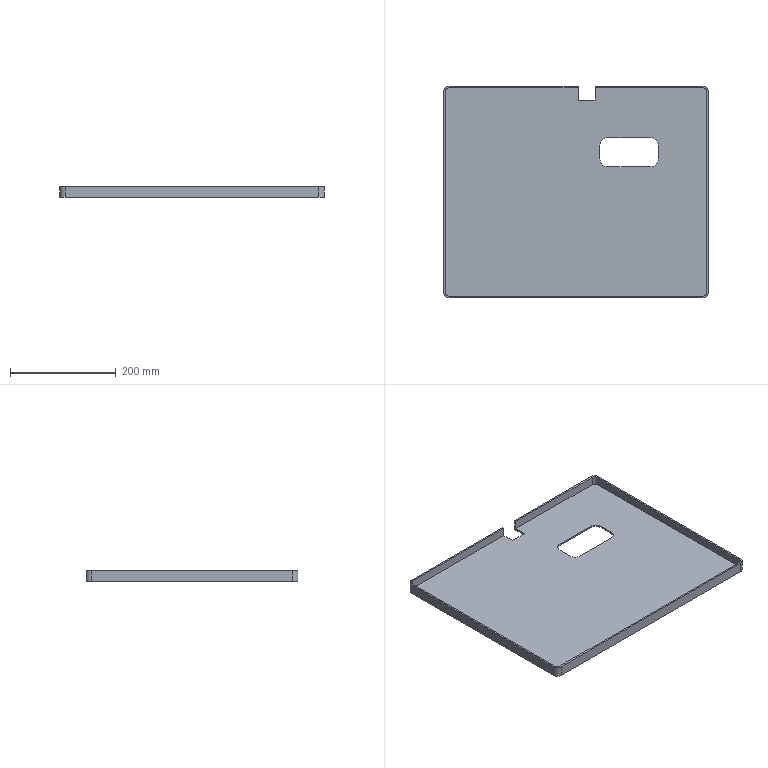Component | SolidWorks | LX-TSJ-16-2 | 1 solid | 32 faces | box 500 x 400 x 20 mm | volume 668381 mm3 | plane 20 | cylinder 12 | commonest cylinder face diameters 20 x4 14 x4 30 x4
STEP:
#1=COLOUR_RGB('',0.7922,0.8196,0.9333);
#2=FILL_AREA_STYLE_COLOUR('',#1);
#3=FILL_AREA_STYLE('',(#2));
#4=SURFACE_STYLE_FILL_AREA(#3);
#5=SURFACE_SIDE_STYLE('',(#4));
#6=SURFACE_STYLE_USAGE(.BOTH.,#5);
#7=PRESENTATION_STYLE_ASSIGNMENT((#6));
#8=CARTESIAN_POINT('',(-5.473,-15.275,-26.153));
#9=VERTEX_POINT('',#8);
#10=CARTESIAN_POINT('',(-5.473,-15.275,-26.823));
#11=VERTEX_POINT('',#10);
#12=CARTESIAN_POINT('',(-5.473,-15.275,-26.153));
#13=DIRECTION('',(0.,0.,-1.));
#14=VECTOR('',#13,39.37);
#15=LINE('',#12,#14);
#16=EDGE_CURVE('',#9,#11,#15,.T.);
#17=ORIENTED_EDGE('',*,*,#16,.F.);
#18=CARTESIAN_POINT('',(-15.08,-15.275,-26.153));
#19=VERTEX_POINT('',#18);
#20=CARTESIAN_POINT('',(-15.08,-15.275,-26.153));
#21=DIRECTION('',(1.,0.,0.));
#22=VECTOR('',#21,39.37);
#23=LINE('',#20,#22);
#24=EDGE_CURVE('',#19,#9,#23,.T.);
#25=ORIENTED_EDGE('',*,*,#24,.F.);
#26=CARTESIAN_POINT('',(-15.08,-15.275,-26.823));
#27=VERTEX_POINT('',#26);
#28=CARTESIAN_POINT('',(-15.08,-15.275,-26.153));
#29=DIRECTION('',(0.,0.,-1.));
#30=VECTOR('',#29,39.37);
#31=LINE('',#28,#30);
#32=EDGE_CURVE('',#19,#27,#31,.T.);
#33=ORIENTED_EDGE('',*,*,#32,.T.);
#34=CARTESIAN_POINT('',(-15.08,-15.275,-26.823));
#35=DIRECTION('',(1.,0.,0.));
#36=VECTOR('',#35,39.37);
#37=LINE('',#34,#36);
#38=EDGE_CURVE('',#27,#11,#37,.T.);
#39=ORIENTED_EDGE('',*,*,#38,.T.);
#40=EDGE_LOOP('',(#17,#25,#33,#39));
#41=FACE_OUTER_BOUND('',#40,.T.);
#42=CARTESIAN_POINT('',(-15.08,-15.275,-26.153));
#43=DIRECTION('',(0.,-1.,0.));
#44=DIRECTION('',(0.,0.,-1.));
#45=AXIS2_PLACEMENT_3D('',#42,#43,#44);
#46=PLANE('',#45);
#47=ADVANCED_FACE('',(#41),#46,.T.);
#48=CARTESIAN_POINT('',(-5.473,-15.157,-26.153));
#49=VERTEX_POINT('',#48);
#50=CARTESIAN_POINT('',(-15.08,-15.157,-26.153));
#51=VERTEX_POINT('',#50);
#52=CARTESIAN_POINT('',(-15.08,-15.157,-26.153));
#53=DIRECTION('',(-1.,0.,0.));
#54=VECTOR('',#53,39.37);
#55=LINE('',#52,#54);
#56=EDGE_CURVE('',#49,#51,#55,.T.);
#57=ORIENTED_EDGE('',*,*,#56,.F.);
#58=CARTESIAN_POINT('',(-5.473,-15.157,-26.941));
#59=VERTEX_POINT('',#58);
#60=CARTESIAN_POINT('',(-5.473,-15.157,-26.153));
#61=DIRECTION('',(0.,0.,-1.));
#62=VECTOR('',#61,39.37);
#63=LINE('',#60,#62);
#64=EDGE_CURVE('',#49,#59,#63,.T.);
#65=ORIENTED_EDGE('',*,*,#64,.T.);
#66=CARTESIAN_POINT('',(-15.08,-15.157,-26.941));
#67=VERTEX_POINT('',#66);
#68=CARTESIAN_POINT('',(-15.08,-15.157,-26.941));
#69=DIRECTION('',(-1.,0.,0.));
#70=VECTOR('',#69,39.37);
#71=LINE('',#68,#70);
#72=EDGE_CURVE('',#59,#67,#71,.T.);
#73=ORIENTED_EDGE('',*,*,#72,.T.);
#74=CARTESIAN_POINT('',(-15.08,-15.157,-26.153));
#75=DIRECTION('',(0.,0.,-1.));
#76=VECTOR('',#75,39.37);
#77=LINE('',#74,#76);
#78=EDGE_CURVE('',#51,#67,#77,.T.);
#79=ORIENTED_EDGE('',*,*,#78,.F.);
#80=EDGE_LOOP('',(#57,#65,#73,#79));
#81=FACE_OUTER_BOUND('',#80,.T.);
#82=CARTESIAN_POINT('',(-15.08,-15.157,-26.153));
#83=DIRECTION('',(0.,-1.,0.));
#84=DIRECTION('',(0.,0.,-1.));
#85=AXIS2_PLACEMENT_3D('',#82,#83,#84);
#86=PLANE('',#85);
#87=ADVANCED_FACE('',(#81),#86,.F.);
#88=ORIENTED_EDGE('',*,*,#72,.F.);
#89=CARTESIAN_POINT('',(-5.473,-16.18,-26.941));
#90=VERTEX_POINT('',#89);
#91=CARTESIAN_POINT('',(-5.473,-30.511,-26.941));
#92=DIRECTION('',(0.,-1.,0.));
#93=VECTOR('',#92,39.37);
#94=LINE('',#91,#93);
#95=EDGE_CURVE('',#59,#90,#94,.T.);
#96=ORIENTED_EDGE('',*,*,#95,.T.);
#97=CARTESIAN_POINT('',(-4.213,-16.18,-26.941));
#98=VERTEX_POINT('',#97);
#99=CARTESIAN_POINT('',(-15.08,-16.18,-26.941));
#100=DIRECTION('',(1.,0.,0.));
#101=VECTOR('',#100,39.37);
#102=LINE('',#99,#101);
#103=EDGE_CURVE('',#90,#98,#102,.T.);
#104=ORIENTED_EDGE('',*,*,#103,.T.);
#105=CARTESIAN_POINT('',(-4.213,-15.157,-26.941));
#106=VERTEX_POINT('',#105);
#107=CARTESIAN_POINT('',(-4.213,-30.511,-26.941));
#108=DIRECTION('',(0.,1.,0.));
#109=VECTOR('',#108,39.37);
#110=LINE('',#107,#109);
#111=EDGE_CURVE('',#98,#106,#110,.T.);
#112=ORIENTED_EDGE('',*,*,#111,.T.);
#113=CARTESIAN_POINT('',(3.818,-15.157,-26.941));
#114=VERTEX_POINT('',#113);
#115=CARTESIAN_POINT('',(-15.08,-15.157,-26.941));
#116=DIRECTION('',(-1.,0.,0.));
#117=VECTOR('',#116,39.37);
#118=LINE('',#115,#117);
#119=EDGE_CURVE('',#114,#106,#118,.T.);
#120=ORIENTED_EDGE('',*,*,#119,.F.);
#121=CARTESIAN_POINT('',(4.212,-15.55,-26.941));
#122=VERTEX_POINT('',#121);
#123=CARTESIAN_POINT('',(3.818,-15.55,-26.941));
#124=DIRECTION('',(0.,0.,1.));
#125=DIRECTION('',(-1.,0.,0.));
#126=AXIS2_PLACEMENT_3D('',#123,#124,#125);
#127=CIRCLE('',#126,0.3937);
#128=EDGE_CURVE('',#122,#114,#127,.T.);
#129=ORIENTED_EDGE('',*,*,#128,.F.);
#130=CARTESIAN_POINT('',(4.212,-30.511,-26.941));
#131=VERTEX_POINT('',#130);
#132=CARTESIAN_POINT('',(4.212,-30.511,-26.941));
#133=DIRECTION('',(0.,1.,0.));
#134=VECTOR('',#133,39.37);
#135=LINE('',#132,#134);
#136=EDGE_CURVE('',#131,#122,#135,.T.);
#137=ORIENTED_EDGE('',*,*,#136,.F.);
#138=CARTESIAN_POINT('',(3.818,-30.905,-26.941));
#139=VERTEX_POINT('',#138);
#140=CARTESIAN_POINT('',(3.818,-30.511,-26.941));
#141=DIRECTION('',(0.,0.,1.));
#142=DIRECTION('',(-1.,0.,0.));
#143=AXIS2_PLACEMENT_3D('',#140,#141,#142);
#144=CIRCLE('',#143,0.3937);
#145=EDGE_CURVE('',#139,#131,#144,.T.);
#146=ORIENTED_EDGE('',*,*,#145,.F.);
#147=CARTESIAN_POINT('',(-15.08,-30.905,-26.941));
#148=VERTEX_POINT('',#147);
#149=CARTESIAN_POINT('',(-15.08,-30.905,-26.941));
#150=DIRECTION('',(1.,0.,0.));
#151=VECTOR('',#150,39.37);
#152=LINE('',#149,#151);
#153=EDGE_CURVE('',#148,#139,#152,.T.);
#154=ORIENTED_EDGE('',*,*,#153,.F.);
#155=CARTESIAN_POINT('',(-15.473,-30.511,-26.941));
#156=VERTEX_POINT('',#155);
#157=CARTESIAN_POINT('',(-15.08,-30.511,-26.941));
#158=DIRECTION('',(0.,0.,1.));
#159=DIRECTION('',(-1.,0.,0.));
#160=AXIS2_PLACEMENT_3D('',#157,#158,#159);
#161=CIRCLE('',#160,0.3937);
#162=EDGE_CURVE('',#156,#148,#161,.T.);
#163=ORIENTED_EDGE('',*,*,#162,.F.);
#164=CARTESIAN_POINT('',(-15.473,-15.55,-26.941));
#165=VERTEX_POINT('',#164);
#166=CARTESIAN_POINT('',(-15.473,-30.511,-26.941));
#167=DIRECTION('',(0.,-1.,0.));
#168=VECTOR('',#167,39.37);
#169=LINE('',#166,#168);
#170=EDGE_CURVE('',#165,#156,#169,.T.);
#171=ORIENTED_EDGE('',*,*,#170,.F.);
#172=CARTESIAN_POINT('',(-15.08,-15.55,-26.941));
#173=DIRECTION('',(0.,0.,1.));
#174=DIRECTION('',(-1.,0.,0.));
#175=AXIS2_PLACEMENT_3D('',#172,#173,#174);
#176=CIRCLE('',#175,0.3937);
#177=EDGE_CURVE('',#67,#165,#176,.T.);
#178=ORIENTED_EDGE('',*,*,#177,.F.);
#179=EDGE_LOOP('',(#88,#96,#104,#112,#120,#129,#137,#146,#154,#163,#171,#178));
#180=FACE_OUTER_BOUND('',#179,.T.);
#181=CARTESIAN_POINT('',(-3.848,-19.572,-26.941));
#182=VERTEX_POINT('',#181);
#183=CARTESIAN_POINT('',(-3.848,-20.563,-26.941));
#184=VERTEX_POINT('',#183);
#185=CARTESIAN_POINT('',(-3.848,-30.511,-26.941));
#186=DIRECTION('',(0.,-1.,0.));
#187=VECTOR('',#186,39.37);
#188=LINE('',#185,#187);
#189=EDGE_CURVE('',#182,#184,#188,.T.);
#190=ORIENTED_EDGE('',*,*,#189,.T.);
#191=CARTESIAN_POINT('',(-3.258,-21.153,-26.941));
#192=VERTEX_POINT('',#191);
#193=CARTESIAN_POINT('',(-3.258,-20.563,-26.941));
#194=DIRECTION('',(0.,0.,1.));
#195=DIRECTION('',(1.,0.,0.));
#196=AXIS2_PLACEMENT_3D('',#193,#194,#195);
#197=CIRCLE('',#196,0.5906);
#198=EDGE_CURVE('',#184,#192,#197,.T.);
#199=ORIENTED_EDGE('',*,*,#198,.T.);
#200=CARTESIAN_POINT('',(-0.09565,-21.153,-26.941));
#201=VERTEX_POINT('',#200);
#202=CARTESIAN_POINT('',(-15.08,-21.153,-26.941));
#203=DIRECTION('',(1.,0.,0.));
#204=VECTOR('',#203,39.37);
#205=LINE('',#202,#204);
#206=EDGE_CURVE('',#192,#201,#205,.T.);
#207=ORIENTED_EDGE('',*,*,#206,.T.);
#208=CARTESIAN_POINT('',(0.4949,-20.563,-26.941));
#209=VERTEX_POINT('',#208);
#210=CARTESIAN_POINT('',(-0.09565,-20.563,-26.941));
#211=DIRECTION('',(0.,0.,1.));
#212=DIRECTION('',(1.,0.,0.));
#213=AXIS2_PLACEMENT_3D('',#210,#211,#212);
#214=CIRCLE('',#213,0.5906);
#215=EDGE_CURVE('',#201,#209,#214,.T.);
#216=ORIENTED_EDGE('',*,*,#215,.T.);
#217=CARTESIAN_POINT('',(0.4949,-19.572,-26.941));
#218=VERTEX_POINT('',#217);
#219=CARTESIAN_POINT('',(0.4949,-30.511,-26.941));
#220=DIRECTION('',(0.,1.,0.));
#221=VECTOR('',#220,39.37);
#222=LINE('',#219,#221);
#223=EDGE_CURVE('',#209,#218,#222,.T.);
#224=ORIENTED_EDGE('',*,*,#223,.T.);
#225=CARTESIAN_POINT('',(-0.09565,-18.981,-26.941));
#226=VERTEX_POINT('',#225);
#227=CARTESIAN_POINT('',(-0.09565,-19.572,-26.941));
#228=DIRECTION('',(0.,0.,1.));
#229=DIRECTION('',(1.,0.,0.));
#230=AXIS2_PLACEMENT_3D('',#227,#228,#229);
#231=CIRCLE('',#230,0.5906);
#232=EDGE_CURVE('',#218,#226,#231,.T.);
#233=ORIENTED_EDGE('',*,*,#232,.T.);
#234=CARTESIAN_POINT('',(-3.258,-18.981,-26.941));
#235=VERTEX_POINT('',#234);
#236=CARTESIAN_POINT('',(-15.08,-18.981,-26.941));
#237=DIRECTION('',(-1.,0.,0.));
#238=VECTOR('',#237,39.37);
#239=LINE('',#236,#238);
#240=EDGE_CURVE('',#226,#235,#239,.T.);
#241=ORIENTED_EDGE('',*,*,#240,.T.);
#242=CARTESIAN_POINT('',(-3.258,-19.572,-26.941));
#243=DIRECTION('',(0.,0.,1.));
#244=DIRECTION('',(1.,0.,0.));
#245=AXIS2_PLACEMENT_3D('',#242,#243,#244);
#246=CIRCLE('',#245,0.5906);
#247=EDGE_CURVE('',#235,#182,#246,.T.);
#248=ORIENTED_EDGE('',*,*,#247,.T.);
#249=EDGE_LOOP('',(#190,#199,#207,#216,#224,#233,#241,#248));
#250=FACE_BOUND('',#249,.T.);
#251=CARTESIAN_POINT('',(-15.08,-30.511,-26.941));
#252=DIRECTION('',(0.,0.,1.));
#253=DIRECTION('',(1.,0.,0.));
#254=AXIS2_PLACEMENT_3D('',#251,#252,#253);
#255=PLANE('',#254);
#256=ADVANCED_FACE('',(#180,#250),#255,.F.);
#257=CARTESIAN_POINT('',(-15.08,-30.905,-26.153));
#258=VERTEX_POINT('',#257);
#259=CARTESIAN_POINT('',(-15.473,-30.511,-26.153));
#260=VERTEX_POINT('',#259);
#261=CARTESIAN_POINT('',(-15.08,-30.511,-26.153));
#262=DIRECTION('',(0.,0.,-1.));
#263=DIRECTION('',(-1.,0.,0.));
#264=AXIS2_PLACEMENT_3D('',#261,#262,#263);
#265=CIRCLE('',#264,0.3937);
#266=EDGE_CURVE('',#258,#260,#265,.T.);
#267=ORIENTED_EDGE('',*,*,#266,.T.);
#268=CARTESIAN_POINT('',(-15.473,-30.511,-26.153));
#269=DIRECTION('',(0.,0.,-1.));
#270=VECTOR('',#269,39.37);
#271=LINE('',#268,#270);
#272=EDGE_CURVE('',#260,#156,#271,.T.);
#273=ORIENTED_EDGE('',*,*,#272,.T.);
#274=ORIENTED_EDGE('',*,*,#162,.T.);
#275=CARTESIAN_POINT('',(-15.08,-30.905,-26.153));
#276=DIRECTION('',(0.,0.,1.));
#277=VECTOR('',#276,39.37);
#278=LINE('',#275,#277);
#279=EDGE_CURVE('',#148,#258,#278,.T.);
#280=ORIENTED_EDGE('',*,*,#279,.T.);
#281=EDGE_LOOP('',(#267,#273,#274,#280));
#282=FACE_OUTER_BOUND('',#281,.T.);
#283=CARTESIAN_POINT('',(-15.08,-30.511,-26.153));
#284=DIRECTION('',(0.,0.,-1.));
#285=DIRECTION('',(-1.,0.,0.));
#286=AXIS2_PLACEMENT_3D('',#283,#284,#285);
#287=CYLINDRICAL_SURFACE('',#286,0.3937);
#288=ADVANCED_FACE('',(#282),#287,.T.);
#289=ORIENTED_EDGE('',*,*,#272,.F.);
#290=CARTESIAN_POINT('',(-15.473,-15.55,-26.153));
#291=VERTEX_POINT('',#290);
#292=CARTESIAN_POINT('',(-15.473,-15.55,-26.153));
#293=DIRECTION('',(0.,-1.,0.));
#294=VECTOR('',#293,39.37);
#295=LINE('',#292,#294);
#296=EDGE_CURVE('',#291,#260,#295,.T.);
#297=ORIENTED_EDGE('',*,*,#296,.F.);
#298=CARTESIAN_POINT('',(-15.473,-15.55,-26.153));
#299=DIRECTION('',(0.,0.,1.));
#300=VECTOR('',#299,39.37);
#301=LINE('',#298,#300);
#302=EDGE_CURVE('',#165,#291,#301,.T.);
#303=ORIENTED_EDGE('',*,*,#302,.F.);
#304=ORIENTED_EDGE('',*,*,#170,.T.);
#305=EDGE_LOOP('',(#289,#297,#303,#304));
#306=FACE_OUTER_BOUND('',#305,.T.);
#307=CARTESIAN_POINT('',(-15.473,-15.55,-26.153));
#308=DIRECTION('',(1.,0.,0.));
#309=DIRECTION('',(-0.,1.,0.));
#310=AXIS2_PLACEMENT_3D('',#307,#308,#309);
#311=PLANE('',#310);
#312=ADVANCED_FACE('',(#306),#311,.F.);
#313=CARTESIAN_POINT('',(-15.08,-15.55,-26.153));
#314=DIRECTION('',(0.,0.,-1.));
#315=DIRECTION('',(-1.,0.,0.));
#316=AXIS2_PLACEMENT_3D('',#313,#314,#315);
#317=CIRCLE('',#316,0.3937);
#318=EDGE_CURVE('',#291,#51,#317,.T.);
#319=ORIENTED_EDGE('',*,*,#318,.T.);
#320=ORIENTED_EDGE('',*,*,#78,.T.);
#321=ORIENTED_EDGE('',*,*,#177,.T.);
#322=ORIENTED_EDGE('',*,*,#302,.T.);
#323=EDGE_LOOP('',(#319,#320,#321,#322));
#324=FACE_OUTER_BOUND('',#323,.T.);
#325=CARTESIAN_POINT('',(-15.08,-15.55,-26.153));
#326=DIRECTION('',(0.,0.,-1.));
#327=DIRECTION('',(-1.,0.,0.));
#328=AXIS2_PLACEMENT_3D('',#325,#326,#327);
#329=CYLINDRICAL_SURFACE('',#328,0.3937);
#330=ADVANCED_FACE('',(#324),#329,.T.);
#331=ORIENTED_EDGE('',*,*,#119,.T.);
#332=CARTESIAN_POINT('',(-4.213,-15.157,-26.153));
#333=VERTEX_POINT('',#332);
#334=CARTESIAN_POINT('',(-4.213,-15.157,-26.153));
#335=DIRECTION('',(0.,0.,1.));
#336=VECTOR('',#335,39.37);
#337=LINE('',#334,#336);
#338=EDGE_CURVE('',#106,#333,#337,.T.);
#339=ORIENTED_EDGE('',*,*,#338,.T.);
#340=CARTESIAN_POINT('',(3.818,-15.157,-26.153));
#341=VERTEX_POINT('',#340);
#342=CARTESIAN_POINT('',(-15.08,-15.157,-26.153));
#343=DIRECTION('',(-1.,0.,0.));
#344=VECTOR('',#343,39.37);
#345=LINE('',#342,#344);
#346=EDGE_CURVE('',#341,#333,#345,.T.);
#347=ORIENTED_EDGE('',*,*,#346,.F.);
#348=CARTESIAN_POINT('',(3.818,-15.157,-26.153));
#349=DIRECTION('',(0.,0.,1.));
#350=VECTOR('',#349,39.37);
#351=LINE('',#348,#350);
#352=EDGE_CURVE('',#114,#341,#351,.T.);
#353=ORIENTED_EDGE('',*,*,#352,.F.);
#354=EDGE_LOOP('',(#331,#339,#347,#353));
#355=FACE_OUTER_BOUND('',#354,.T.);
#356=CARTESIAN_POINT('',(-15.08,-15.157,-26.153));
#357=DIRECTION('',(0.,-1.,0.));
#358=DIRECTION('',(0.,0.,-1.));
#359=AXIS2_PLACEMENT_3D('',#356,#357,#358);
#360=PLANE('',#359);
#361=ADVANCED_FACE('',(#355),#360,.F.);
#362=CARTESIAN_POINT('',(4.212,-15.55,-26.153));
#363=VERTEX_POINT('',#362);
#364=CARTESIAN_POINT('',(3.818,-15.55,-26.153));
#365=DIRECTION('',(0.,0.,-1.));
#366=DIRECTION('',(-1.,0.,0.));
#367=AXIS2_PLACEMENT_3D('',#364,#365,#366);
#368=CIRCLE('',#367,0.3937);
#369=EDGE_CURVE('',#341,#363,#368,.T.);
#370=ORIENTED_EDGE('',*,*,#369,.T.);
#371=CARTESIAN_POINT('',(4.212,-15.55,-26.153));
#372=DIRECTION('',(0.,0.,-1.));
#373=VECTOR('',#372,39.37);
#374=LINE('',#371,#373);
#375=EDGE_CURVE('',#363,#122,#374,.T.);
#376=ORIENTED_EDGE('',*,*,#375,.T.);
#377=ORIENTED_EDGE('',*,*,#128,.T.);
#378=ORIENTED_EDGE('',*,*,#352,.T.);
#379=EDGE_LOOP('',(#370,#376,#377,#378));
#380=FACE_OUTER_BOUND('',#379,.T.);
#381=CARTESIAN_POINT('',(3.818,-15.55,-26.153));
#382=DIRECTION('',(0.,0.,-1.));
#383=DIRECTION('',(-1.,0.,0.));
#384=AXIS2_PLACEMENT_3D('',#381,#382,#383);
#385=CYLINDRICAL_SURFACE('',#384,0.3937);
#386=ADVANCED_FACE('',(#380),#385,.T.);
#387=ORIENTED_EDGE('',*,*,#375,.F.);
#388=CARTESIAN_POINT('',(4.212,-30.511,-26.153));
#389=VERTEX_POINT('',#388);
#390=CARTESIAN_POINT('',(4.212,-15.55,-26.153));
#391=DIRECTION('',(-0.,1.,0.));
#392=VECTOR('',#391,39.37);
#393=LINE('',#390,#392);
#394=EDGE_CURVE('',#389,#363,#393,.T.);
#395=ORIENTED_EDGE('',*,*,#394,.F.);
#396=CARTESIAN_POINT('',(4.212,-30.511,-26.153));
#397=DIRECTION('',(0.,0.,1.));
#398=VECTOR('',#397,39.37);
#399=LINE('',#396,#398);
#400=EDGE_CURVE('',#131,#389,#399,.T.);
#401=ORIENTED_EDGE('',*,*,#400,.F.);
#402=ORIENTED_EDGE('',*,*,#136,.T.);
#403=EDGE_LOOP('',(#387,#395,#401,#402));
#404=FACE_OUTER_BOUND('',#403,.T.);
#405=CARTESIAN_POINT('',(4.212,-15.55,-26.153));
#406=DIRECTION('',(-1.,-0.,0.));
#407=DIRECTION('',(0.,-1.,0.));
#408=AXIS2_PLACEMENT_3D('',#405,#406,#407);
#409=PLANE('',#408);
#410=ADVANCED_FACE('',(#404),#409,.F.);
#411=CARTESIAN_POINT('',(3.818,-30.905,-26.153));
#412=VERTEX_POINT('',#411);
#413=CARTESIAN_POINT('',(3.818,-30.511,-26.153));
#414=DIRECTION('',(0.,0.,-1.));
#415=DIRECTION('',(-1.,0.,0.));
#416=AXIS2_PLACEMENT_3D('',#413,#414,#415);
#417=CIRCLE('',#416,0.3937);
#418=EDGE_CURVE('',#389,#412,#417,.T.);
#419=ORIENTED_EDGE('',*,*,#418,.T.);
#420=CARTESIAN_POINT('',(3.818,-30.905,-26.153));
#421=DIRECTION('',(0.,0.,-1.));
#422=VECTOR('',#421,39.37);
#423=LINE('',#420,#422);
#424=EDGE_CURVE('',#412,#139,#423,.T.);
#425=ORIENTED_EDGE('',*,*,#424,.T.);
#426=ORIENTED_EDGE('',*,*,#145,.T.);
#427=ORIENTED_EDGE('',*,*,#400,.T.);
#428=EDGE_LOOP('',(#419,#425,#426,#427));
#429=FACE_OUTER_BOUND('',#428,.T.);
#430=CARTESIAN_POINT('',(3.818,-30.511,-26.153));
#431=DIRECTION('',(0.,0.,-1.));
#432=DIRECTION('',(-1.,0.,0.));
#433=AXIS2_PLACEMENT_3D('',#430,#431,#432);
#434=CYLINDRICAL_SURFACE('',#433,0.3937);
#435=ADVANCED_FACE('',(#429),#434,.T.);
#436=ORIENTED_EDGE('',*,*,#424,.F.);
#437=CARTESIAN_POINT('',(-15.08,-30.905,-26.153));
#438=DIRECTION('',(1.,0.,0.));
#439=VECTOR('',#438,39.37);
#440=LINE('',#437,#439);
#441=EDGE_CURVE('',#258,#412,#440,.T.);
#442=ORIENTED_EDGE('',*,*,#441,.F.);
#443=ORIENTED_EDGE('',*,*,#279,.F.);
#444=ORIENTED_EDGE('',*,*,#153,.T.);
#445=EDGE_LOOP('',(#436,#442,#443,#444));
#446=FACE_OUTER_BOUND('',#445,.T.);
#447=CARTESIAN_POINT('',(-15.08,-30.905,-26.153));
#448=DIRECTION('',(0.,1.,0.));
#449=DIRECTION('',(0.,0.,1.));
#450=AXIS2_PLACEMENT_3D('',#447,#448,#449);
#451=PLANE('',#450);
#452=ADVANCED_FACE('',(#446),#451,.F.);
#453=CARTESIAN_POINT('',(-5.473,-16.18,-26.153));
#454=DIRECTION('',(0.,-1.,0.));
#455=VECTOR('',#454,39.37);
#456=LINE('',#453,#455);
#457=EDGE_CURVE('',#49,#9,#456,.T.);
#458=ORIENTED_EDGE('',*,*,#457,.F.);
#459=ORIENTED_EDGE('',*,*,#56,.T.);
#460=ORIENTED_EDGE('',*,*,#318,.F.);
#461=ORIENTED_EDGE('',*,*,#296,.T.);
#462=ORIENTED_EDGE('',*,*,#266,.F.);
#463=ORIENTED_EDGE('',*,*,#441,.T.);
#464=ORIENTED_EDGE('',*,*,#418,.F.);
#465=ORIENTED_EDGE('',*,*,#394,.T.);
#466=ORIENTED_EDGE('',*,*,#369,.F.);
#467=ORIENTED_EDGE('',*,*,#346,.T.);
#468=CARTESIAN_POINT('',(-4.213,-15.275,-26.153));
#469=VERTEX_POINT('',#468);
#470=CARTESIAN_POINT('',(-4.213,-16.18,-26.153));
#471=DIRECTION('',(0.,1.,0.));
#472=VECTOR('',#471,39.37);
#473=LINE('',#470,#472);
#474=EDGE_CURVE('',#469,#333,#473,.T.);
#475=ORIENTED_EDGE('',*,*,#474,.F.);
#476=CARTESIAN_POINT('',(3.818,-15.275,-26.153));
#477=VERTEX_POINT('',#476);
#478=CARTESIAN_POINT('',(-15.08,-15.275,-26.153));
#479=DIRECTION('',(1.,0.,0.));
#480=VECTOR('',#479,39.37);
#481=LINE('',#478,#480);
#482=EDGE_CURVE('',#469,#477,#481,.T.);
#483=ORIENTED_EDGE('',*,*,#482,.T.);
#484=CARTESIAN_POINT('',(4.094,-15.55,-26.153));
#485=VERTEX_POINT('',#484);
#486=CARTESIAN_POINT('',(3.818,-15.55,-26.153));
#487=DIRECTION('',(0.,0.,-1.));
#488=DIRECTION('',(-1.,0.,0.));
#489=AXIS2_PLACEMENT_3D('',#486,#487,#488);
#490=CIRCLE('',#489,0.2756);
#491=EDGE_CURVE('',#477,#485,#490,.T.);
#492=ORIENTED_EDGE('',*,*,#491,.T.);
#493=CARTESIAN_POINT('',(4.094,-30.511,-26.153));
#494=VERTEX_POINT('',#493);
#495=CARTESIAN_POINT('',(4.094,-30.511,-26.153));
#496=DIRECTION('',(0.,-1.,0.));
#497=VECTOR('',#496,39.37);
#498=LINE('',#495,#497);
#499=EDGE_CURVE('',#485,#494,#498,.T.);
#500=ORIENTED_EDGE('',*,*,#499,.T.);
#501=CARTESIAN_POINT('',(3.818,-30.787,-26.153));
#502=VERTEX_POINT('',#501);
#503=CARTESIAN_POINT('',(3.818,-30.511,-26.153));
#504=DIRECTION('',(0.,0.,-1.));
#505=DIRECTION('',(-1.,0.,0.));
#506=AXIS2_PLACEMENT_3D('',#503,#504,#505);
#507=CIRCLE('',#506,0.2756);
#508=EDGE_CURVE('',#494,#502,#507,.T.);
#509=ORIENTED_EDGE('',*,*,#508,.T.);
#510=CARTESIAN_POINT('',(-15.08,-30.787,-26.153));
#511=VERTEX_POINT('',#510);
#512=CARTESIAN_POINT('',(-15.08,-30.787,-26.153));
#513=DIRECTION('',(-1.,0.,0.));
#514=VECTOR('',#513,39.37);
#515=LINE('',#512,#514);
#516=EDGE_CURVE('',#502,#511,#515,.T.);
#517=ORIENTED_EDGE('',*,*,#516,.T.);
#518=CARTESIAN_POINT('',(-15.355,-30.511,-26.153));
#519=VERTEX_POINT('',#518);
#520=CARTESIAN_POINT('',(-15.08,-30.511,-26.153));
#521=DIRECTION('',(0.,0.,-1.));
#522=DIRECTION('',(-1.,0.,0.));
#523=AXIS2_PLACEMENT_3D('',#520,#521,#522);
#524=CIRCLE('',#523,0.2756);
#525=EDGE_CURVE('',#511,#519,#524,.T.);
#526=ORIENTED_EDGE('',*,*,#525,.T.);
#527=CARTESIAN_POINT('',(-15.355,-15.55,-26.153));
#528=VERTEX_POINT('',#527);
#529=CARTESIAN_POINT('',(-15.355,-30.511,-26.153));
#530=DIRECTION('',(0.,1.,0.));
#531=VECTOR('',#530,39.37);
#532=LINE('',#529,#531);
#533=EDGE_CURVE('',#519,#528,#532,.T.);
#534=ORIENTED_EDGE('',*,*,#533,.T.);
#535=CARTESIAN_POINT('',(-15.08,-15.55,-26.153));
#536=DIRECTION('',(0.,0.,-1.));
#537=DIRECTION('',(-1.,0.,0.));
#538=AXIS2_PLACEMENT_3D('',#535,#536,#537);
#539=CIRCLE('',#538,0.2756);
#540=EDGE_CURVE('',#528,#19,#539,.T.);
#541=ORIENTED_EDGE('',*,*,#540,.T.);
#542=ORIENTED_EDGE('',*,*,#24,.T.);
#543=EDGE_LOOP('',(#458,#459,#460,#461,#462,#463,#464,#465,#466,#467,#475,#483,#492,#500,#509,#517,#526,#534,#541,#542));
#544=FACE_OUTER_BOUND('',#543,.T.);
#545=CARTESIAN_POINT('',(-15.08,-30.511,-26.153));
#546=DIRECTION('',(0.,0.,1.));
#547=DIRECTION('',(1.,0.,0.));
#548=AXIS2_PLACEMENT_3D('',#545,#546,#547);
#549=PLANE('',#548);
#550=ADVANCED_FACE('',(#544),#549,.T.);
#551=ORIENTED_EDGE('',*,*,#516,.F.);
#552=CARTESIAN_POINT('',(3.818,-30.787,-26.823));
#553=VERTEX_POINT('',#552);
#554=CARTESIAN_POINT('',(3.818,-30.787,-26.153));
#555=DIRECTION('',(0.,0.,-1.));
#556=VECTOR('',#555,39.37);
#557=LINE('',#554,#556);
#558=EDGE_CURVE('',#502,#553,#557,.T.);
#559=ORIENTED_EDGE('',*,*,#558,.T.);
#560=CARTESIAN_POINT('',(-15.08,-30.787,-26.823));
#561=VERTEX_POINT('',#560);
#562=CARTESIAN_POINT('',(-15.08,-30.787,-26.823));
#563=DIRECTION('',(-1.,0.,0.));
#564=VECTOR('',#563,39.37);
#565=LINE('',#562,#564);
#566=EDGE_CURVE('',#553,#561,#565,.T.);
#567=ORIENTED_EDGE('',*,*,#566,.T.);
#568=CARTESIAN_POINT('',(-15.08,-30.787,-26.153));
#569=DIRECTION('',(0.,0.,1.));
#570=VECTOR('',#569,39.37);
#571=LINE('',#568,#570);
#572=EDGE_CURVE('',#561,#511,#571,.T.);
#573=ORIENTED_EDGE('',*,*,#572,.T.);
#574=EDGE_LOOP('',(#551,#559,#567,#573));
#575=FACE_OUTER_BOUND('',#574,.T.);
#576=CARTESIAN_POINT('',(-15.08,-30.787,-26.153));
#577=DIRECTION('',(0.,1.,0.));
#578=DIRECTION('',(0.,0.,1.));
#579=AXIS2_PLACEMENT_3D('',#576,#577,#578);
#580=PLANE('',#579);
#581=ADVANCED_FACE('',(#575),#580,.T.);
#582=ORIENTED_EDGE('',*,*,#558,.F.);
#583=ORIENTED_EDGE('',*,*,#508,.F.);
#584=CARTESIAN_POINT('',(4.094,-30.511,-26.823));
#585=VERTEX_POINT('',#584);
#586=CARTESIAN_POINT('',(4.094,-30.511,-26.153));
#587=DIRECTION('',(0.,0.,1.));
#588=VECTOR('',#587,39.37);
#589=LINE('',#586,#588);
#590=EDGE_CURVE('',#585,#494,#589,.T.);
#591=ORIENTED_EDGE('',*,*,#590,.F.);
#592=CARTESIAN_POINT('',(3.818,-30.511,-26.823));
#593=DIRECTION('',(0.,0.,1.));
#594=DIRECTION('',(-1.,0.,0.));
#595=AXIS2_PLACEMENT_3D('',#592,#593,#594);
#596=CIRCLE('',#595,0.2756);
#597=EDGE_CURVE('',#553,#585,#596,.T.);
#598=ORIENTED_EDGE('',*,*,#597,.F.);
#599=EDGE_LOOP('',(#582,#583,#591,#598));
#600=FACE_OUTER_BOUND('',#599,.T.);
#601=CARTESIAN_POINT('',(3.818,-30.511,-26.153));
#602=DIRECTION('',(0.,0.,-1.));
#603=DIRECTION('',(-1.,0.,0.));
#604=AXIS2_PLACEMENT_3D('',#601,#602,#603);
#605=CYLINDRICAL_SURFACE('',#604,0.2756);
#606=ADVANCED_FACE('',(#600),#605,.F.);
#607=ORIENTED_EDGE('',*,*,#499,.F.);
#608=CARTESIAN_POINT('',(4.094,-15.55,-26.823));
#609=VERTEX_POINT('',#608);
#610=CARTESIAN_POINT('',(4.094,-15.55,-26.153));
#611=DIRECTION('',(0.,0.,-1.));
#612=VECTOR('',#611,39.37);
#613=LINE('',#610,#612);
#614=EDGE_CURVE('',#485,#609,#613,.T.);
#615=ORIENTED_EDGE('',*,*,#614,.T.);
#616=CARTESIAN_POINT('',(4.094,-15.55,-26.823));
#617=DIRECTION('',(0.,-1.,0.));
#618=VECTOR('',#617,39.37);
#619=LINE('',#616,#618);
#620=EDGE_CURVE('',#609,#585,#619,.T.);
#621=ORIENTED_EDGE('',*,*,#620,.T.);
#622=ORIENTED_EDGE('',*,*,#590,.T.);
#623=EDGE_LOOP('',(#607,#615,#621,#622));
#624=FACE_OUTER_BOUND('',#623,.T.);
#625=CARTESIAN_POINT('',(4.094,-15.55,-26.153));
#626=DIRECTION('',(-1.,-0.,0.));
#627=DIRECTION('',(0.,-1.,0.));
#628=AXIS2_PLACEMENT_3D('',#625,#626,#627);
#629=PLANE('',#628);
#630=ADVANCED_FACE('',(#624),#629,.T.);
#631=ORIENTED_EDGE('',*,*,#614,.F.);
#632=ORIENTED_EDGE('',*,*,#491,.F.);
#633=CARTESIAN_POINT('',(3.818,-15.275,-26.823));
#634=VERTEX_POINT('',#633);
#635=CARTESIAN_POINT('',(3.818,-15.275,-26.153));
#636=DIRECTION('',(0.,0.,1.));
#637=VECTOR('',#636,39.37);
#638=LINE('',#635,#637);
#639=EDGE_CURVE('',#634,#477,#638,.T.);
#640=ORIENTED_EDGE('',*,*,#639,.F.);
#641=CARTESIAN_POINT('',(3.818,-15.55,-26.823));
#642=DIRECTION('',(0.,0.,1.));
#643=DIRECTION('',(-1.,0.,0.));
#644=AXIS2_PLACEMENT_3D('',#641,#642,#643);
#645=CIRCLE('',#644,0.2756);
#646=EDGE_CURVE('',#609,#634,#645,.T.);
#647=ORIENTED_EDGE('',*,*,#646,.F.);
#648=EDGE_LOOP('',(#631,#632,#640,#647));
#649=FACE_OUTER_BOUND('',#648,.T.);
#650=CARTESIAN_POINT('',(3.818,-15.55,-26.153));
#651=DIRECTION('',(0.,0.,-1.));
#652=DIRECTION('',(-1.,0.,0.));
#653=AXIS2_PLACEMENT_3D('',#650,#651,#652);
#654=CYLINDRICAL_SURFACE('',#653,0.2756);
#655=ADVANCED_FACE('',(#649),#654,.F.);
#656=CARTESIAN_POINT('',(-4.213,-15.275,-26.823));
#657=VERTEX_POINT('',#656);
#658=CARTESIAN_POINT('',(-4.213,-15.275,-26.153));
#659=DIRECTION('',(0.,0.,1.));
#660=VECTOR('',#659,39.37);
#661=LINE('',#658,#660);
#662=EDGE_CURVE('',#657,#469,#661,.T.);
#663=ORIENTED_EDGE('',*,*,#662,.F.);
#664=CARTESIAN_POINT('',(-15.08,-15.275,-26.823));
#665=DIRECTION('',(1.,0.,0.));
#666=VECTOR('',#665,39.37);
#667=LINE('',#664,#666);
#668=EDGE_CURVE('',#657,#634,#667,.T.);
#669=ORIENTED_EDGE('',*,*,#668,.T.);
#670=ORIENTED_EDGE('',*,*,#639,.T.);
#671=ORIENTED_EDGE('',*,*,#482,.F.);
#672=EDGE_LOOP('',(#663,#669,#670,#671));
#673=FACE_OUTER_BOUND('',#672,.T.);
#674=CARTESIAN_POINT('',(-15.08,-15.275,-26.153));
#675=DIRECTION('',(0.,-1.,0.));
#676=DIRECTION('',(0.,0.,-1.));
#677=AXIS2_PLACEMENT_3D('',#674,#675,#676);
#678=PLANE('',#677);
#679=ADVANCED_FACE('',(#673),#678,.T.);
#680=ORIENTED_EDGE('',*,*,#32,.F.);
#681=ORIENTED_EDGE('',*,*,#540,.F.);
#682=CARTESIAN_POINT('',(-15.355,-15.55,-26.823));
#683=VERTEX_POINT('',#682);
#684=CARTESIAN_POINT('',(-15.355,-15.55,-26.153));
#685=DIRECTION('',(0.,0.,1.));
#686=VECTOR('',#685,39.37);
#687=LINE('',#684,#686);
#688=EDGE_CURVE('',#683,#528,#687,.T.);
#689=ORIENTED_EDGE('',*,*,#688,.F.);
#690=CARTESIAN_POINT('',(-15.08,-15.55,-26.823));
#691=DIRECTION('',(0.,0.,1.));
#692=DIRECTION('',(-1.,0.,0.));
#693=AXIS2_PLACEMENT_3D('',#690,#691,#692);
#694=CIRCLE('',#693,0.2756);
#695=EDGE_CURVE('',#27,#683,#694,.T.);
#696=ORIENTED_EDGE('',*,*,#695,.F.);
#697=EDGE_LOOP('',(#680,#681,#689,#696));
#698=FACE_OUTER_BOUND('',#697,.T.);
#699=CARTESIAN_POINT('',(-15.08,-15.55,-26.153));
#700=DIRECTION('',(0.,0.,-1.));
#701=DIRECTION('',(-1.,0.,0.));
#702=AXIS2_PLACEMENT_3D('',#699,#700,#701);
#703=CYLINDRICAL_SURFACE('',#702,0.2756);
#704=ADVANCED_FACE('',(#698),#703,.F.);
#705=ORIENTED_EDGE('',*,*,#533,.F.);
#706=CARTESIAN_POINT('',(-15.355,-30.511,-26.823));
#707=VERTEX_POINT('',#706);
#708=CARTESIAN_POINT('',(-15.355,-30.511,-26.153));
#709=DIRECTION('',(0.,0.,-1.));
#710=VECTOR('',#709,39.37);
#711=LINE('',#708,#710);
#712=EDGE_CURVE('',#519,#707,#711,.T.);
#713=ORIENTED_EDGE('',*,*,#712,.T.);
#714=CARTESIAN_POINT('',(-15.355,-15.55,-26.823));
#715=DIRECTION('',(-0.,1.,0.));
#716=VECTOR('',#715,39.37);
#717=LINE('',#714,#716);
#718=EDGE_CURVE('',#707,#683,#717,.T.);
#719=ORIENTED_EDGE('',*,*,#718,.T.);
#720=ORIENTED_EDGE('',*,*,#688,.T.);
#721=EDGE_LOOP('',(#705,#713,#719,#720));
#722=FACE_OUTER_BOUND('',#721,.T.);
#723=CARTESIAN_POINT('',(-15.355,-15.55,-26.153));
#724=DIRECTION('',(1.,0.,0.));
#725=DIRECTION('',(-0.,1.,0.));
#726=AXIS2_PLACEMENT_3D('',#723,#724,#725);
#727=PLANE('',#726);
#728=ADVANCED_FACE('',(#722),#727,.T.);
#729=ORIENTED_EDGE('',*,*,#712,.F.);
#730=ORIENTED_EDGE('',*,*,#525,.F.);
#731=ORIENTED_EDGE('',*,*,#572,.F.);
#732=CARTESIAN_POINT('',(-15.08,-30.511,-26.823));
#733=DIRECTION('',(0.,0.,1.));
#734=DIRECTION('',(-1.,0.,0.));
#735=AXIS2_PLACEMENT_3D('',#732,#733,#734);
#736=CIRCLE('',#735,0.2756);
#737=EDGE_CURVE('',#707,#561,#736,.T.);
#738=ORIENTED_EDGE('',*,*,#737,.F.);
#739=EDGE_LOOP('',(#729,#730,#731,#738));
#740=FACE_OUTER_BOUND('',#739,.T.);
#741=CARTESIAN_POINT('',(-15.08,-30.511,-26.153));
#742=DIRECTION('',(0.,0.,-1.));
#743=DIRECTION('',(-1.,0.,0.));
#744=AXIS2_PLACEMENT_3D('',#741,#742,#743);
#745=CYLINDRICAL_SURFACE('',#744,0.2756);
#746=ADVANCED_FACE('',(#740),#745,.F.);
#747=CARTESIAN_POINT('',(-5.473,-16.18,-26.823));
#748=VERTEX_POINT('',#747);
#749=CARTESIAN_POINT('',(-5.473,-30.511,-26.823));
#750=DIRECTION('',(0.,-1.,0.));
#751=VECTOR('',#750,39.37);
#752=LINE('',#749,#751);
#753=EDGE_CURVE('',#11,#748,#752,.T.);
#754=ORIENTED_EDGE('',*,*,#753,.F.);
#755=ORIENTED_EDGE('',*,*,#38,.F.);
#756=ORIENTED_EDGE('',*,*,#695,.T.);
#757=ORIENTED_EDGE('',*,*,#718,.F.);
#758=ORIENTED_EDGE('',*,*,#737,.T.);
#759=ORIENTED_EDGE('',*,*,#566,.F.);
#760=ORIENTED_EDGE('',*,*,#597,.T.);
#761=ORIENTED_EDGE('',*,*,#620,.F.);
#762=ORIENTED_EDGE('',*,*,#646,.T.);
#763=ORIENTED_EDGE('',*,*,#668,.F.);
#764=CARTESIAN_POINT('',(-4.213,-16.18,-26.823));
#765=VERTEX_POINT('',#764);
#766=CARTESIAN_POINT('',(-4.213,-30.511,-26.823));
#767=DIRECTION('',(0.,1.,0.));
#768=VECTOR('',#767,39.37);
#769=LINE('',#766,#768);
#770=EDGE_CURVE('',#765,#657,#769,.T.);
#771=ORIENTED_EDGE('',*,*,#770,.F.);
#772=CARTESIAN_POINT('',(-15.08,-16.18,-26.823));
#773=DIRECTION('',(1.,0.,0.));
#774=VECTOR('',#773,39.37);
#775=LINE('',#772,#774);
#776=EDGE_CURVE('',#748,#765,#775,.T.);
#777=ORIENTED_EDGE('',*,*,#776,.F.);
#778=EDGE_LOOP('',(#754,#755,#756,#757,#758,#759,#760,#761,#762,#763,#771,#777));
#779=FACE_OUTER_BOUND('',#778,.T.);
#780=CARTESIAN_POINT('',(0.4949,-20.563,-26.823));
#781=VERTEX_POINT('',#780);
#782=CARTESIAN_POINT('',(0.4949,-19.572,-26.823));
#783=VERTEX_POINT('',#782);
#784=CARTESIAN_POINT('',(0.4949,-18.981,-26.823));
#785=DIRECTION('',(0.,1.,0.));
#786=VECTOR('',#785,39.37);
#787=LINE('',#784,#786);
#788=EDGE_CURVE('',#781,#783,#787,.T.);
#789=ORIENTED_EDGE('',*,*,#788,.F.);
#790=CARTESIAN_POINT('',(-0.09565,-21.153,-26.823));
#791=VERTEX_POINT('',#790);
#792=CARTESIAN_POINT('',(-0.09565,-20.563,-26.823));
#793=DIRECTION('',(0.,0.,-1.));
#794=DIRECTION('',(1.,0.,0.));
#795=AXIS2_PLACEMENT_3D('',#792,#793,#794);
#796=CIRCLE('',#795,0.5906);
#797=EDGE_CURVE('',#781,#791,#796,.T.);
#798=ORIENTED_EDGE('',*,*,#797,.T.);
#799=CARTESIAN_POINT('',(-3.258,-21.153,-26.823));
#800=VERTEX_POINT('',#799);
#801=CARTESIAN_POINT('',(-3.848,-21.153,-26.823));
#802=DIRECTION('',(1.,0.,0.));
#803=VECTOR('',#802,39.37);
#804=LINE('',#801,#803);
#805=EDGE_CURVE('',#800,#791,#804,.T.);
#806=ORIENTED_EDGE('',*,*,#805,.F.);
#807=CARTESIAN_POINT('',(-3.848,-20.563,-26.823));
#808=VERTEX_POINT('',#807);
#809=CARTESIAN_POINT('',(-3.258,-20.563,-26.823));
#810=DIRECTION('',(0.,0.,-1.));
#811=DIRECTION('',(1.,0.,0.));
#812=AXIS2_PLACEMENT_3D('',#809,#810,#811);
#813=CIRCLE('',#812,0.5906);
#814=EDGE_CURVE('',#800,#808,#813,.T.);
#815=ORIENTED_EDGE('',*,*,#814,.T.);
#816=CARTESIAN_POINT('',(-3.848,-19.572,-26.823));
#817=VERTEX_POINT('',#816);
#818=CARTESIAN_POINT('',(-3.848,-18.981,-26.823));
#819=DIRECTION('',(0.,-1.,0.));
#820=VECTOR('',#819,39.37);
#821=LINE('',#818,#820);
#822=EDGE_CURVE('',#817,#808,#821,.T.);
#823=ORIENTED_EDGE('',*,*,#822,.F.);
#824=CARTESIAN_POINT('',(-3.258,-18.981,-26.823));
#825=VERTEX_POINT('',#824);
#826=CARTESIAN_POINT('',(-3.258,-19.572,-26.823));
#827=DIRECTION('',(0.,0.,-1.));
#828=DIRECTION('',(1.,0.,0.));
#829=AXIS2_PLACEMENT_3D('',#826,#827,#828);
#830=CIRCLE('',#829,0.5906);
#831=EDGE_CURVE('',#817,#825,#830,.T.);
#832=ORIENTED_EDGE('',*,*,#831,.T.);
#833=CARTESIAN_POINT('',(-0.09565,-18.981,-26.823));
#834=VERTEX_POINT('',#833);
#835=CARTESIAN_POINT('',(-3.848,-18.981,-26.823));
#836=DIRECTION('',(-1.,0.,0.));
#837=VECTOR('',#836,39.37);
#838=LINE('',#835,#837);
#839=EDGE_CURVE('',#834,#825,#838,.T.);
#840=ORIENTED_EDGE('',*,*,#839,.F.);
#841=CARTESIAN_POINT('',(-0.09565,-19.572,-26.823));
#842=DIRECTION('',(0.,0.,-1.));
#843=DIRECTION('',(1.,0.,0.));
#844=AXIS2_PLACEMENT_3D('',#841,#842,#843);
#845=CIRCLE('',#844,0.5906);
#846=EDGE_CURVE('',#834,#783,#845,.T.);
#847=ORIENTED_EDGE('',*,*,#846,.T.);
#848=EDGE_LOOP('',(#789,#798,#806,#815,#823,#832,#840,#847));
#849=FACE_BOUND('',#848,.T.);
#850=CARTESIAN_POINT('',(-15.08,-30.511,-26.823));
#851=DIRECTION('',(0.,0.,1.));
#852=DIRECTION('',(1.,0.,0.));
#853=AXIS2_PLACEMENT_3D('',#850,#851,#852);
#854=PLANE('',#853);
#855=ADVANCED_FACE('',(#779,#849),#854,.T.);
#856=ORIENTED_EDGE('',*,*,#223,.F.);
#857=CARTESIAN_POINT('',(0.4949,-20.563,-26.823));
#858=DIRECTION('',(0.,0.,1.));
#859=VECTOR('',#858,39.37);
#860=LINE('',#857,#859);
#861=EDGE_CURVE('',#209,#781,#860,.T.);
#862=ORIENTED_EDGE('',*,*,#861,.T.);
#863=ORIENTED_EDGE('',*,*,#788,.T.);
#864=CARTESIAN_POINT('',(0.4949,-19.572,-26.941));
#865=DIRECTION('',(0.,0.,-1.));
#866=VECTOR('',#865,39.37);
#867=LINE('',#864,#866);
#868=EDGE_CURVE('',#783,#218,#867,.T.);
#869=ORIENTED_EDGE('',*,*,#868,.T.);
#870=EDGE_LOOP('',(#856,#862,#863,#869));
#871=FACE_OUTER_BOUND('',#870,.T.);
#872=CARTESIAN_POINT('',(0.4949,-18.981,-31.783));
#873=DIRECTION('',(1.,0.,0.));
#874=DIRECTION('',(0.,0.,-1.));
#875=AXIS2_PLACEMENT_3D('',#872,#873,#874);
#876=PLANE('',#875);
#877=ADVANCED_FACE('',(#871),#876,.F.);
#878=ORIENTED_EDGE('',*,*,#805,.T.);
#879=CARTESIAN_POINT('',(-0.09565,-21.153,-26.941));
#880=DIRECTION('',(0.,0.,-1.));
#881=VECTOR('',#880,39.37);
#882=LINE('',#879,#881);
#883=EDGE_CURVE('',#791,#201,#882,.T.);
#884=ORIENTED_EDGE('',*,*,#883,.T.);
#885=ORIENTED_EDGE('',*,*,#206,.F.);
#886=CARTESIAN_POINT('',(-3.258,-21.153,-26.823));
#887=DIRECTION('',(0.,0.,1.));
#888=VECTOR('',#887,39.37);
#889=LINE('',#886,#888);
#890=EDGE_CURVE('',#192,#800,#889,.T.);
#891=ORIENTED_EDGE('',*,*,#890,.T.);
#892=EDGE_LOOP('',(#878,#884,#885,#891));
#893=FACE_OUTER_BOUND('',#892,.T.);
#894=CARTESIAN_POINT('',(-3.848,-21.153,-31.783));
#895=DIRECTION('',(0.,-1.,0.));
#896=DIRECTION('',(0.,0.,-1.));
#897=AXIS2_PLACEMENT_3D('',#894,#895,#896);
#898=PLANE('',#897);
#899=ADVANCED_FACE('',(#893),#898,.F.);
#900=ORIENTED_EDGE('',*,*,#189,.F.);
#901=CARTESIAN_POINT('',(-3.848,-19.572,-26.823));
#902=DIRECTION('',(0.,0.,1.));
#903=VECTOR('',#902,39.37);
#904=LINE('',#901,#903);
#905=EDGE_CURVE('',#182,#817,#904,.T.);
#906=ORIENTED_EDGE('',*,*,#905,.T.);
#907=ORIENTED_EDGE('',*,*,#822,.T.);
#908=CARTESIAN_POINT('',(-3.848,-20.563,-26.941));
#909=DIRECTION('',(0.,0.,-1.));
#910=VECTOR('',#909,39.37);
#911=LINE('',#908,#910);
#912=EDGE_CURVE('',#808,#184,#911,.T.);
#913=ORIENTED_EDGE('',*,*,#912,.T.);
#914=EDGE_LOOP('',(#900,#906,#907,#913));
#915=FACE_OUTER_BOUND('',#914,.T.);
#916=CARTESIAN_POINT('',(-3.848,-18.981,-31.783));
#917=DIRECTION('',(-1.,0.,0.));
#918=DIRECTION('',(0.,0.,1.));
#919=AXIS2_PLACEMENT_3D('',#916,#917,#918);
#920=PLANE('',#919);
#921=ADVANCED_FACE('',(#915),#920,.F.);
#922=ORIENTED_EDGE('',*,*,#839,.T.);
#923=CARTESIAN_POINT('',(-3.258,-18.981,-26.941));
#924=DIRECTION('',(0.,0.,-1.));
#925=VECTOR('',#924,39.37);
#926=LINE('',#923,#925);
#927=EDGE_CURVE('',#825,#235,#926,.T.);
#928=ORIENTED_EDGE('',*,*,#927,.T.);
#929=ORIENTED_EDGE('',*,*,#240,.F.);
#930=CARTESIAN_POINT('',(-0.09565,-18.981,-26.823));
#931=DIRECTION('',(0.,0.,1.));
#932=VECTOR('',#931,39.37);
#933=LINE('',#930,#932);
#934=EDGE_CURVE('',#226,#834,#933,.T.);
#935=ORIENTED_EDGE('',*,*,#934,.T.);
#936=EDGE_LOOP('',(#922,#928,#929,#935));
#937=FACE_OUTER_BOUND('',#936,.T.);
#938=CARTESIAN_POINT('',(-3.848,-18.981,-31.783));
#939=DIRECTION('',(0.,1.,0.));
#940=DIRECTION('',(0.,0.,1.));
#941=AXIS2_PLACEMENT_3D('',#938,#939,#940);
#942=PLANE('',#941);
#943=ADVANCED_FACE('',(#937),#942,.F.);
#944=ORIENTED_EDGE('',*,*,#247,.F.);
#945=ORIENTED_EDGE('',*,*,#927,.F.);
#946=ORIENTED_EDGE('',*,*,#831,.F.);
#947=ORIENTED_EDGE('',*,*,#905,.F.);
#948=EDGE_LOOP('',(#944,#945,#946,#947));
#949=FACE_OUTER_BOUND('',#948,.T.);
#950=CARTESIAN_POINT('',(-3.258,-19.572,-31.783));
#951=DIRECTION('',(0.,0.,-1.));
#952=DIRECTION('',(-1.,0.,0.));
#953=AXIS2_PLACEMENT_3D('',#950,#951,#952);
#954=CYLINDRICAL_SURFACE('',#953,0.5906);
#955=ADVANCED_FACE('',(#949),#954,.F.);
#956=ORIENTED_EDGE('',*,*,#215,.F.);
#957=ORIENTED_EDGE('',*,*,#883,.F.);
#958=ORIENTED_EDGE('',*,*,#797,.F.);
#959=ORIENTED_EDGE('',*,*,#861,.F.);
#960=EDGE_LOOP('',(#956,#957,#958,#959));
#961=FACE_OUTER_BOUND('',#960,.T.);
#962=CARTESIAN_POINT('',(-0.09565,-20.563,-31.783));
#963=DIRECTION('',(0.,0.,-1.));
#964=DIRECTION('',(-1.,0.,0.));
#965=AXIS2_PLACEMENT_3D('',#962,#963,#964);
#966=CYLINDRICAL_SURFACE('',#965,0.5906);
#967=ADVANCED_FACE('',(#961),#966,.F.);
#968=ORIENTED_EDGE('',*,*,#198,.F.);
#969=ORIENTED_EDGE('',*,*,#912,.F.);
#970=ORIENTED_EDGE('',*,*,#814,.F.);
#971=ORIENTED_EDGE('',*,*,#890,.F.);
#972=EDGE_LOOP('',(#968,#969,#970,#971));
#973=FACE_OUTER_BOUND('',#972,.T.);
#974=CARTESIAN_POINT('',(-3.258,-20.563,-31.783));
#975=DIRECTION('',(0.,0.,-1.));
#976=DIRECTION('',(-1.,0.,0.));
#977=AXIS2_PLACEMENT_3D('',#974,#975,#976);
#978=CYLINDRICAL_SURFACE('',#977,0.5906);
#979=ADVANCED_FACE('',(#973),#978,.F.);
#980=ORIENTED_EDGE('',*,*,#232,.F.);
#981=ORIENTED_EDGE('',*,*,#868,.F.);
#982=ORIENTED_EDGE('',*,*,#846,.F.);
#983=ORIENTED_EDGE('',*,*,#934,.F.);
#984=EDGE_LOOP('',(#980,#981,#982,#983));
#985=FACE_OUTER_BOUND('',#984,.T.);
#986=CARTESIAN_POINT('',(-0.09565,-19.572,-31.783));
#987=DIRECTION('',(0.,0.,-1.));
#988=DIRECTION('',(-1.,0.,0.));
#989=AXIS2_PLACEMENT_3D('',#986,#987,#988);
#990=CYLINDRICAL_SURFACE('',#989,0.5906);
#991=ADVANCED_FACE('',(#985),#990,.F.);
#992=ORIENTED_EDGE('',*,*,#753,.T.);
#993=CARTESIAN_POINT('',(-5.473,-16.18,-26.941));
#994=DIRECTION('',(0.,0.,1.));
#995=VECTOR('',#994,39.37);
#996=LINE('',#993,#995);
#997=EDGE_CURVE('',#90,#748,#996,.T.);
#998=ORIENTED_EDGE('',*,*,#997,.F.);
#999=ORIENTED_EDGE('',*,*,#95,.F.);
#1000=ORIENTED_EDGE('',*,*,#64,.F.);
#1001=ORIENTED_EDGE('',*,*,#457,.T.);
#1002=ORIENTED_EDGE('',*,*,#16,.T.);
#1003=EDGE_LOOP('',(#992,#998,#999,#1000,#1001,#1002));
#1004=FACE_OUTER_BOUND('',#1003,.T.);
#1005=CARTESIAN_POINT('',(-5.473,-16.18,-26.941));
#1006=DIRECTION('',(-1.,0.,0.));
#1007=DIRECTION('',(0.,0.,1.));
#1008=AXIS2_PLACEMENT_3D('',#1005,#1006,#1007);
#1009=PLANE('',#1008);
#1010=ADVANCED_FACE('',(#1004),#1009,.F.);
#1011=ORIENTED_EDGE('',*,*,#770,.T.);
#1012=ORIENTED_EDGE('',*,*,#662,.T.);
#1013=ORIENTED_EDGE('',*,*,#474,.T.);
#1014=ORIENTED_EDGE('',*,*,#338,.F.);
#1015=ORIENTED_EDGE('',*,*,#111,.F.);
#1016=CARTESIAN_POINT('',(-4.213,-16.18,-26.941));
#1017=DIRECTION('',(0.,0.,1.));
#1018=VECTOR('',#1017,39.37);
#1019=LINE('',#1016,#1018);
#1020=EDGE_CURVE('',#98,#765,#1019,.T.);
#1021=ORIENTED_EDGE('',*,*,#1020,.T.);
#1022=EDGE_LOOP('',(#1011,#1012,#1013,#1014,#1015,#1021));
#1023=FACE_OUTER_BOUND('',#1022,.T.);
#1024=CARTESIAN_POINT('',(-4.213,-16.18,-26.941));
#1025=DIRECTION('',(1.,0.,0.));
#1026=DIRECTION('',(0.,0.,-1.));
#1027=AXIS2_PLACEMENT_3D('',#1024,#1025,#1026);
#1028=PLANE('',#1027);
#1029=ADVANCED_FACE('',(#1023),#1028,.F.);
#1030=ORIENTED_EDGE('',*,*,#776,.T.);
#1031=ORIENTED_EDGE('',*,*,#1020,.F.);
#1032=ORIENTED_EDGE('',*,*,#103,.F.);
#1033=ORIENTED_EDGE('',*,*,#997,.T.);
#1034=EDGE_LOOP('',(#1030,#1031,#1032,#1033));
#1035=FACE_OUTER_BOUND('',#1034,.T.);
#1036=CARTESIAN_POINT('',(-5.473,-16.18,-26.941));
#1037=DIRECTION('',(0.,-1.,0.));
#1038=DIRECTION('',(0.,0.,-1.));
#1039=AXIS2_PLACEMENT_3D('',#1036,#1037,#1038);
#1040=PLANE('',#1039);
#1041=ADVANCED_FACE('',(#1035),#1040,.F.);
#1042=CLOSED_SHELL('',(#47,#87,#256,#288,#312,#330,#361,#386,#410,#435,#452,#550,#581,#606,#630,#655,#679,#704,#728,#746,#855,#877,#899,#921,#943,#955,#967,#979,#991,#1010,#1029,#1041));
#1043=MANIFOLD_SOLID_BREP('',#1042);
#1044=STYLED_ITEM('',(#7),#1043);
#1045=PRESENTATION_LAYER_ASSIGNMENT('','',(#1044));
#1046=CARTESIAN_POINT('',(0.,0.,0.));
#1047=DIRECTION('',(0.,0.,1.));
#1048=DIRECTION('',(1.,0.,0.));
#1049=AXIS2_PLACEMENT_3D('',#1046,#1047,#1048);
#1050=(LENGTH_UNIT()NAMED_UNIT(*)SI_UNIT($,.METRE.));
#1051=LENGTH_MEASURE_WITH_UNIT(LENGTH_MEASURE(0.0254),#1050);
#1052=DIMENSIONAL_EXPONENTS(1.,0.,0.,0.,0.,0.,0.);
#1053=(CONVERSION_BASED_UNIT('',#1051)LENGTH_UNIT()NAMED_UNIT(#1052));
#1054=UNCERTAINTY_MEASURE_WITH_UNIT(LENGTH_MEASURE(0.00001),#1053,'','');
#1055=(NAMED_UNIT(*)PLANE_ANGLE_UNIT()SI_UNIT($,.RADIAN.));
#1056=(NAMED_UNIT(*)SI_UNIT($,.STERADIAN.)SOLID_ANGLE_UNIT());
#1057=(GEOMETRIC_REPRESENTATION_CONTEXT(3)GLOBAL_UNCERTAINTY_ASSIGNED_CONTEXT((#1054))GLOBAL_UNIT_ASSIGNED_CONTEXT((#1053,#1055,#1056))REPRESENTATION_CONTEXT('',''));
#1058=ADVANCED_BREP_SHAPE_REPRESENTATION('',(#1043,#1049),#1057);
#1059=(LENGTH_UNIT()NAMED_UNIT(*)SI_UNIT($,.METRE.));
#1060=LENGTH_MEASURE_WITH_UNIT(LENGTH_MEASURE(0.0254),#1059);
#1061=DIMENSIONAL_EXPONENTS(1.,0.,0.,0.,0.,0.,0.);
#1062=(CONVERSION_BASED_UNIT('',#1060)LENGTH_UNIT()NAMED_UNIT(#1061));
#1063=UNCERTAINTY_MEASURE_WITH_UNIT(LENGTH_MEASURE(0.00001),#1062,'','');
#1064=(NAMED_UNIT(*)PLANE_ANGLE_UNIT()SI_UNIT($,.RADIAN.));
#1065=(NAMED_UNIT(*)SI_UNIT($,.STERADIAN.)SOLID_ANGLE_UNIT());
#1066=(GEOMETRIC_REPRESENTATION_CONTEXT(3)GLOBAL_UNCERTAINTY_ASSIGNED_CONTEXT((#1063))GLOBAL_UNIT_ASSIGNED_CONTEXT((#1062,#1064,#1065))REPRESENTATION_CONTEXT('',''));
#1067=MECHANICAL_DESIGN_GEOMETRIC_PRESENTATION_REPRESENTATION('',(#1044),#1066);